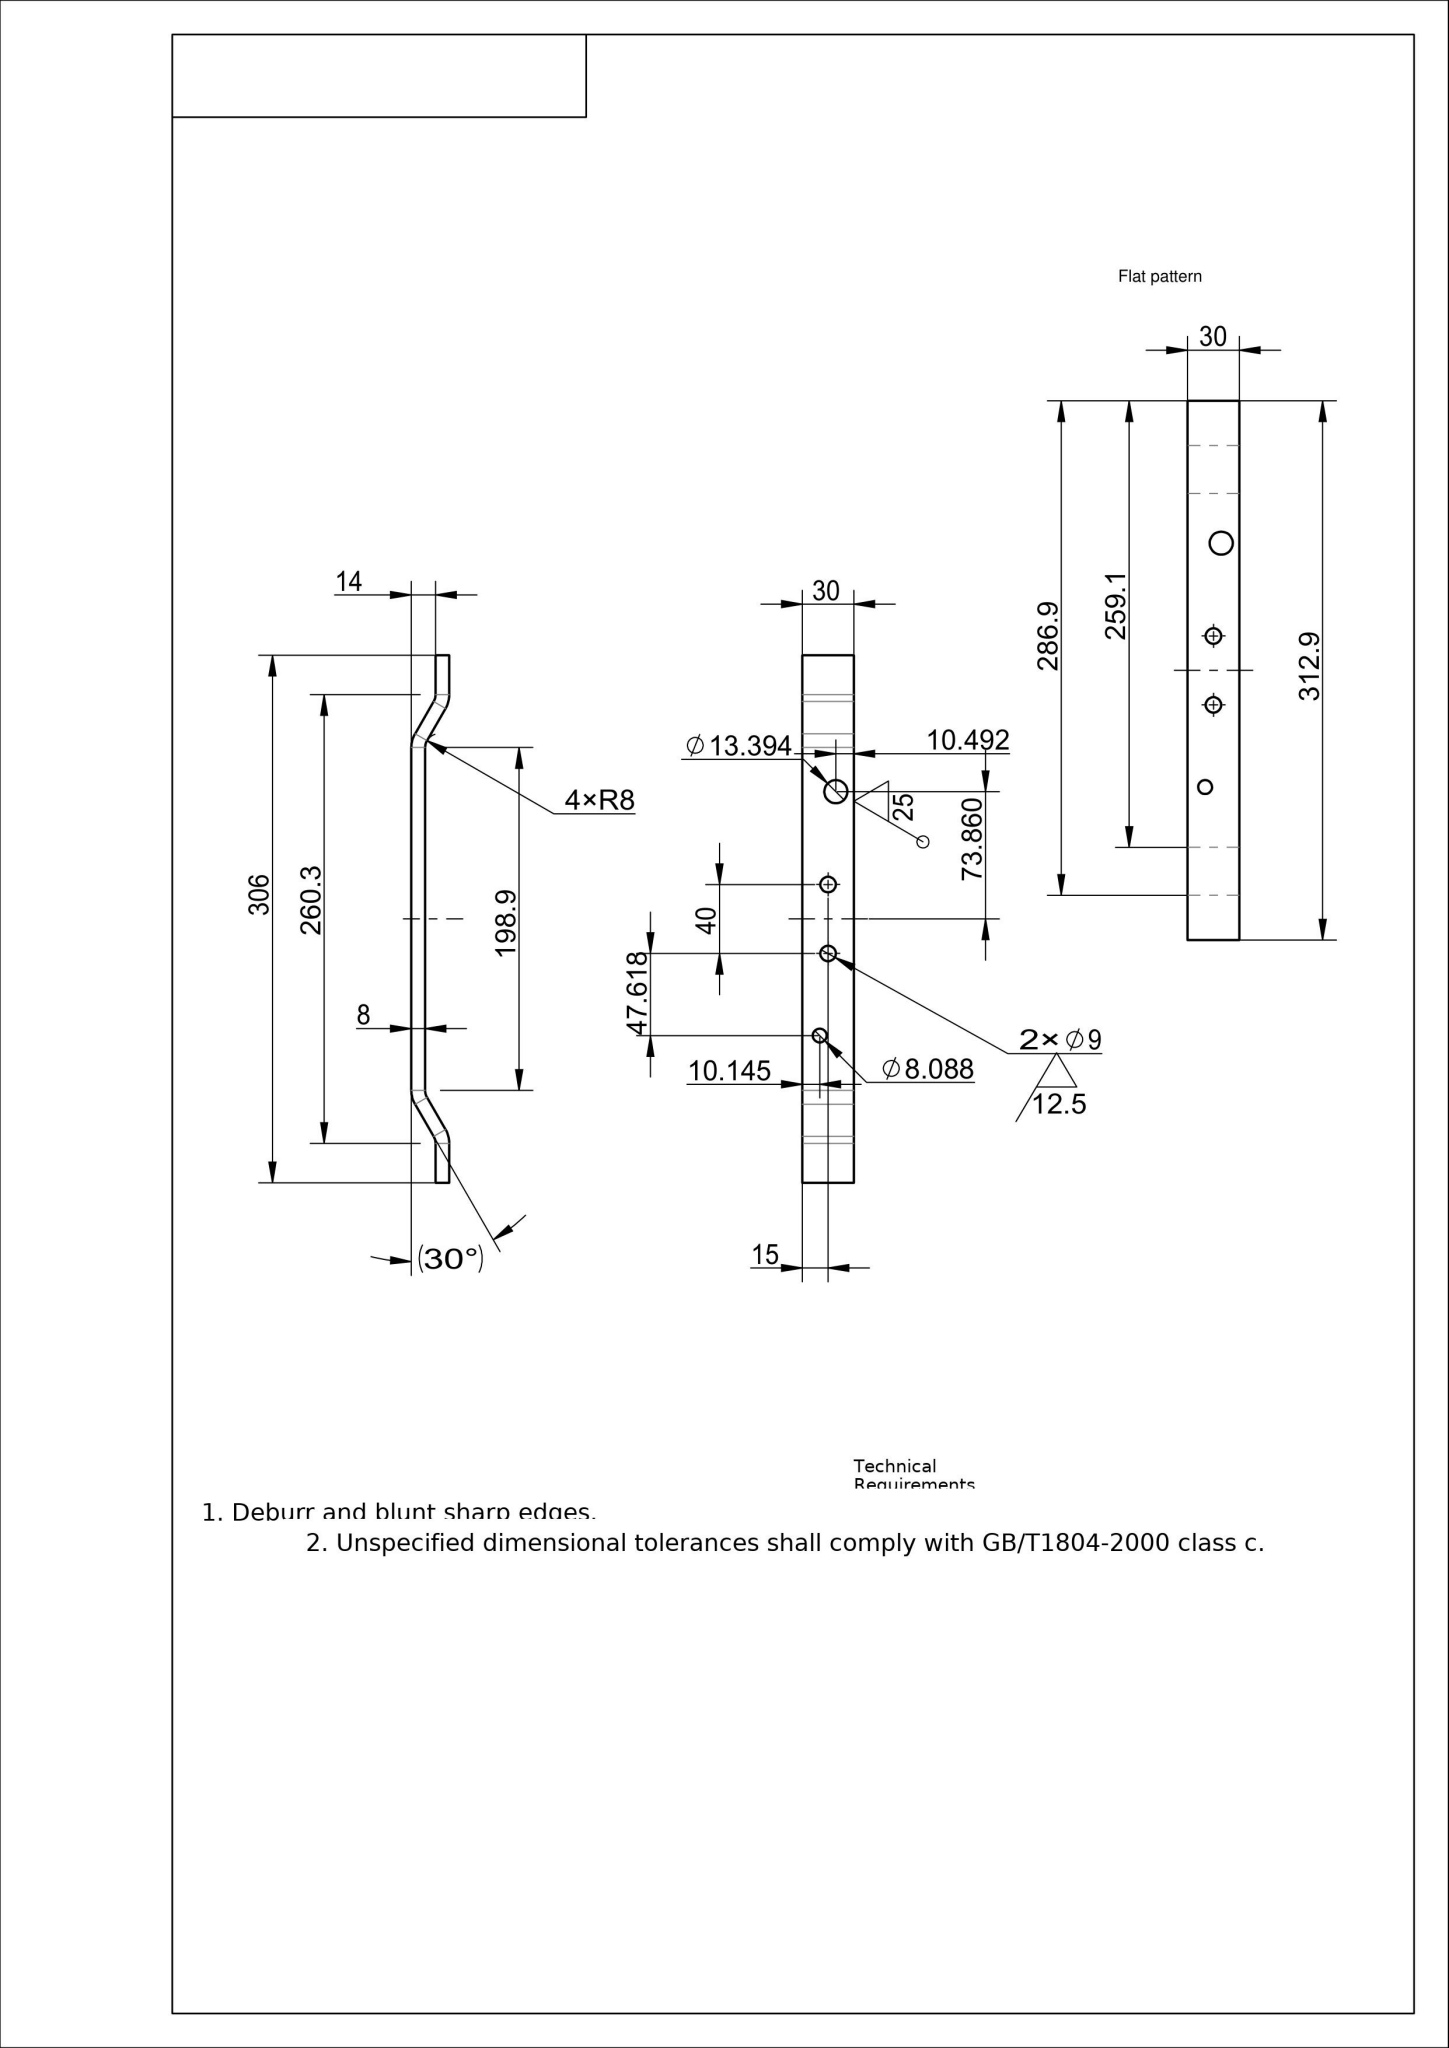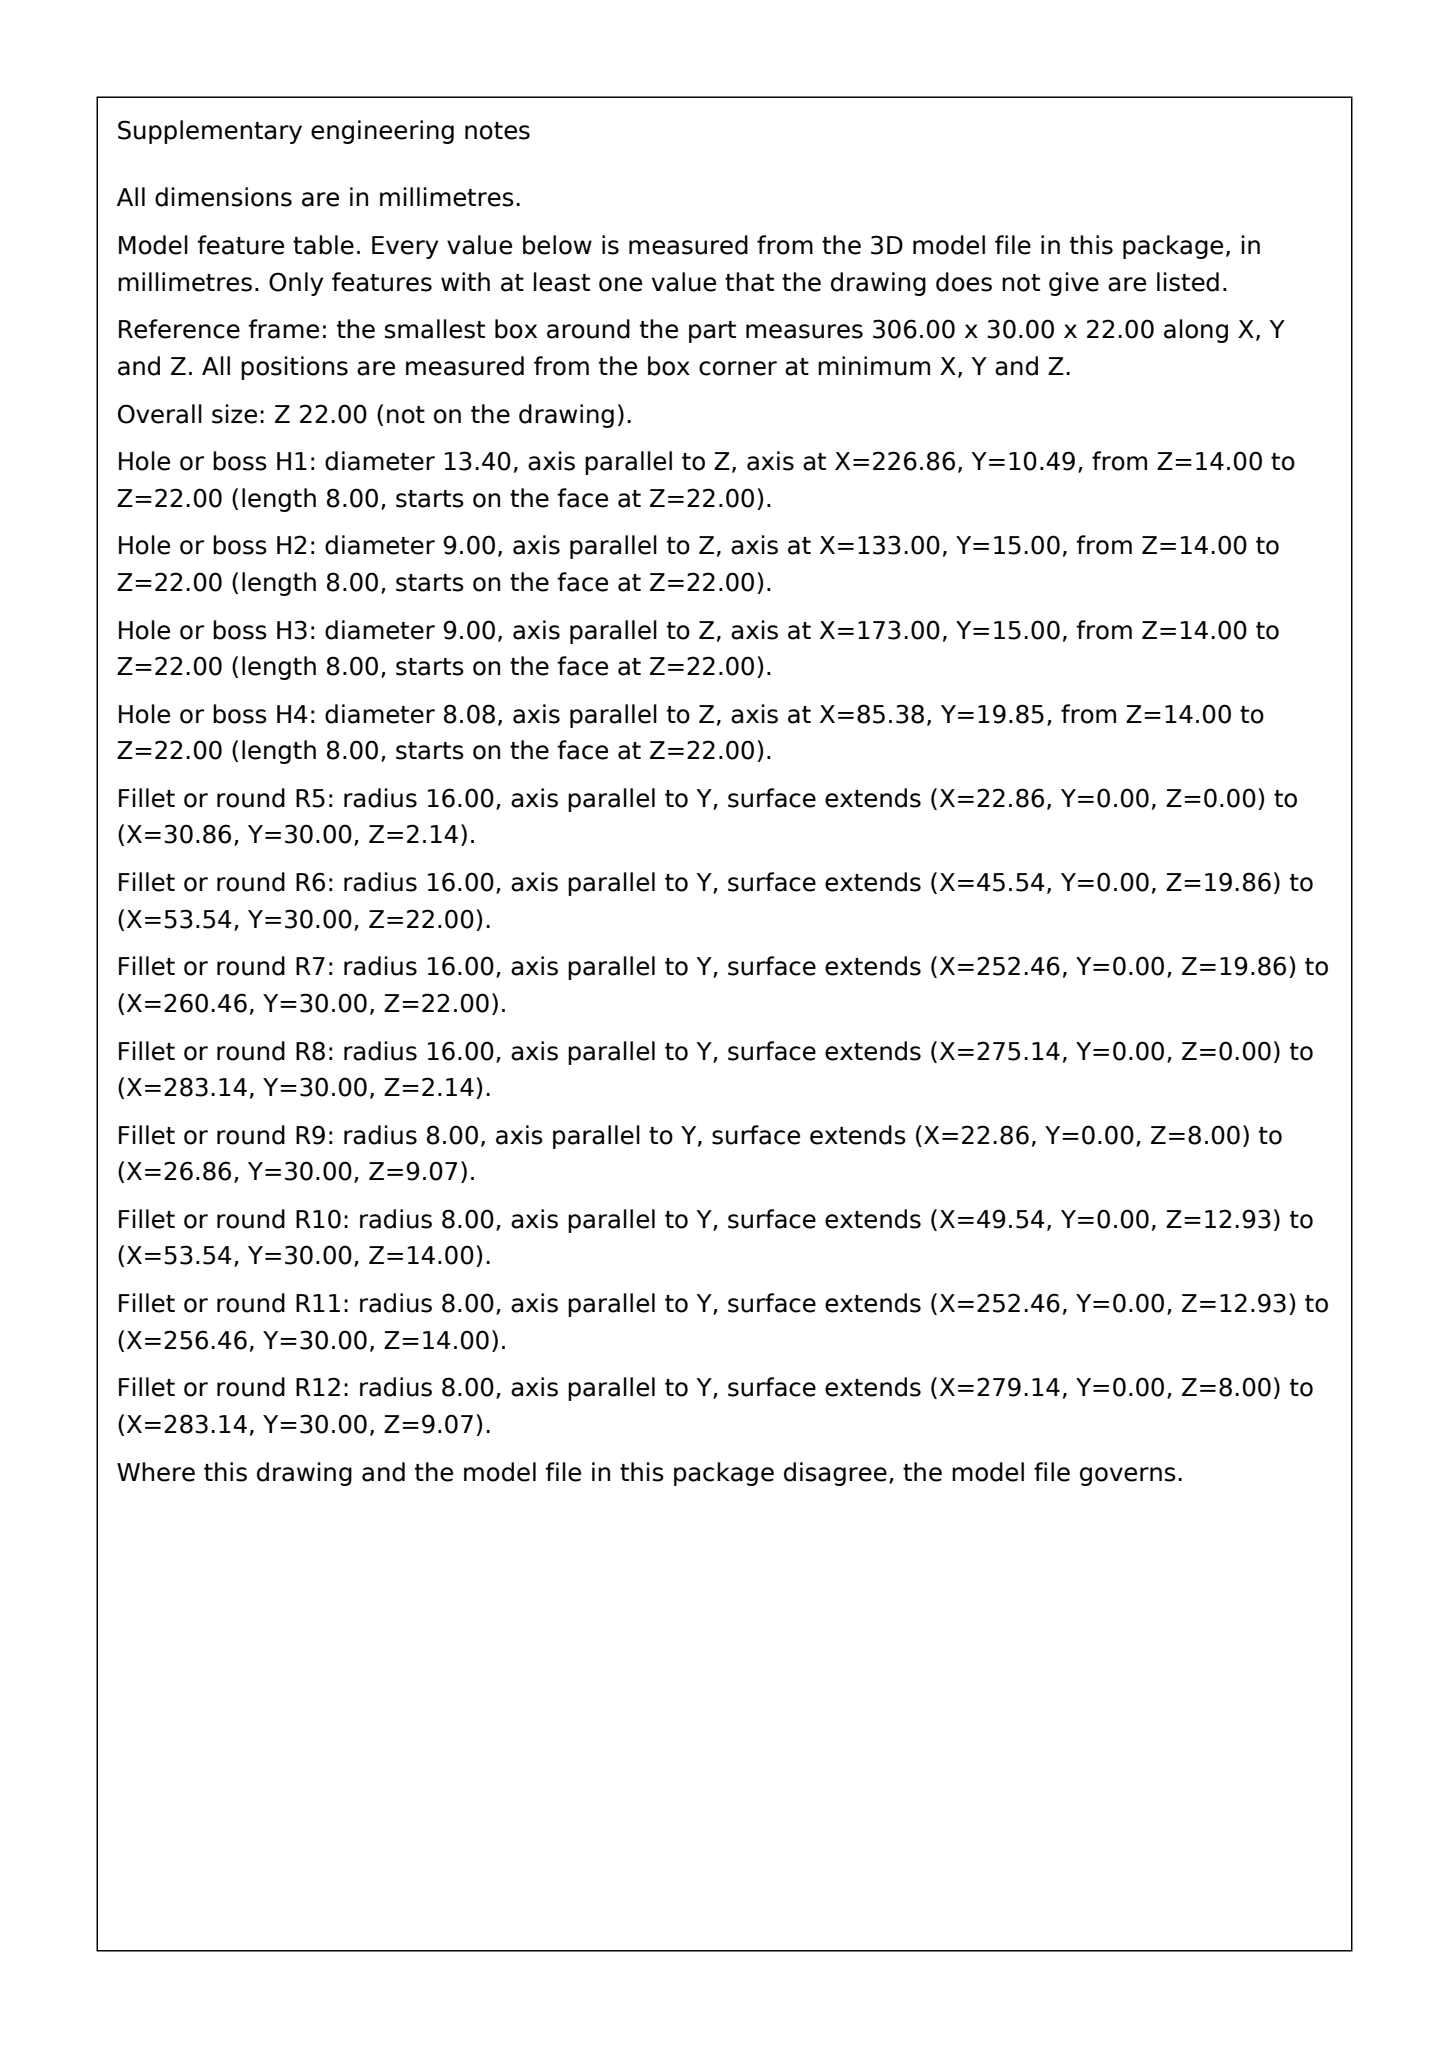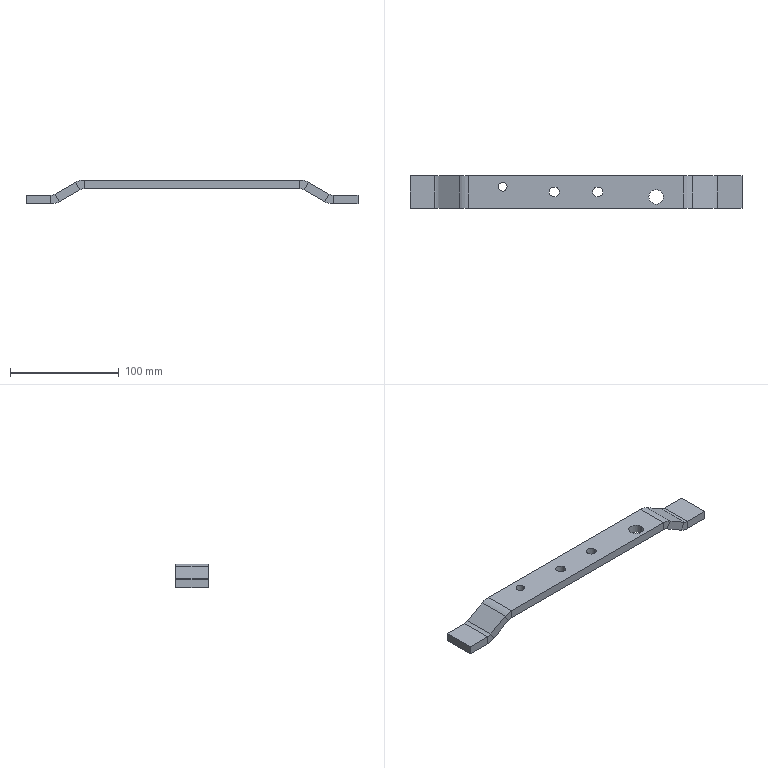Part | SolidWorks | mm | 1 solid | 46 faces | box 306 x 30 x 22 mm | volume 72543 mm3 | plane 30 | cylinder 16 | commonest cylinder face diameters 9 x4 16 x4 32 x4 8.088 x2 13.394 x2